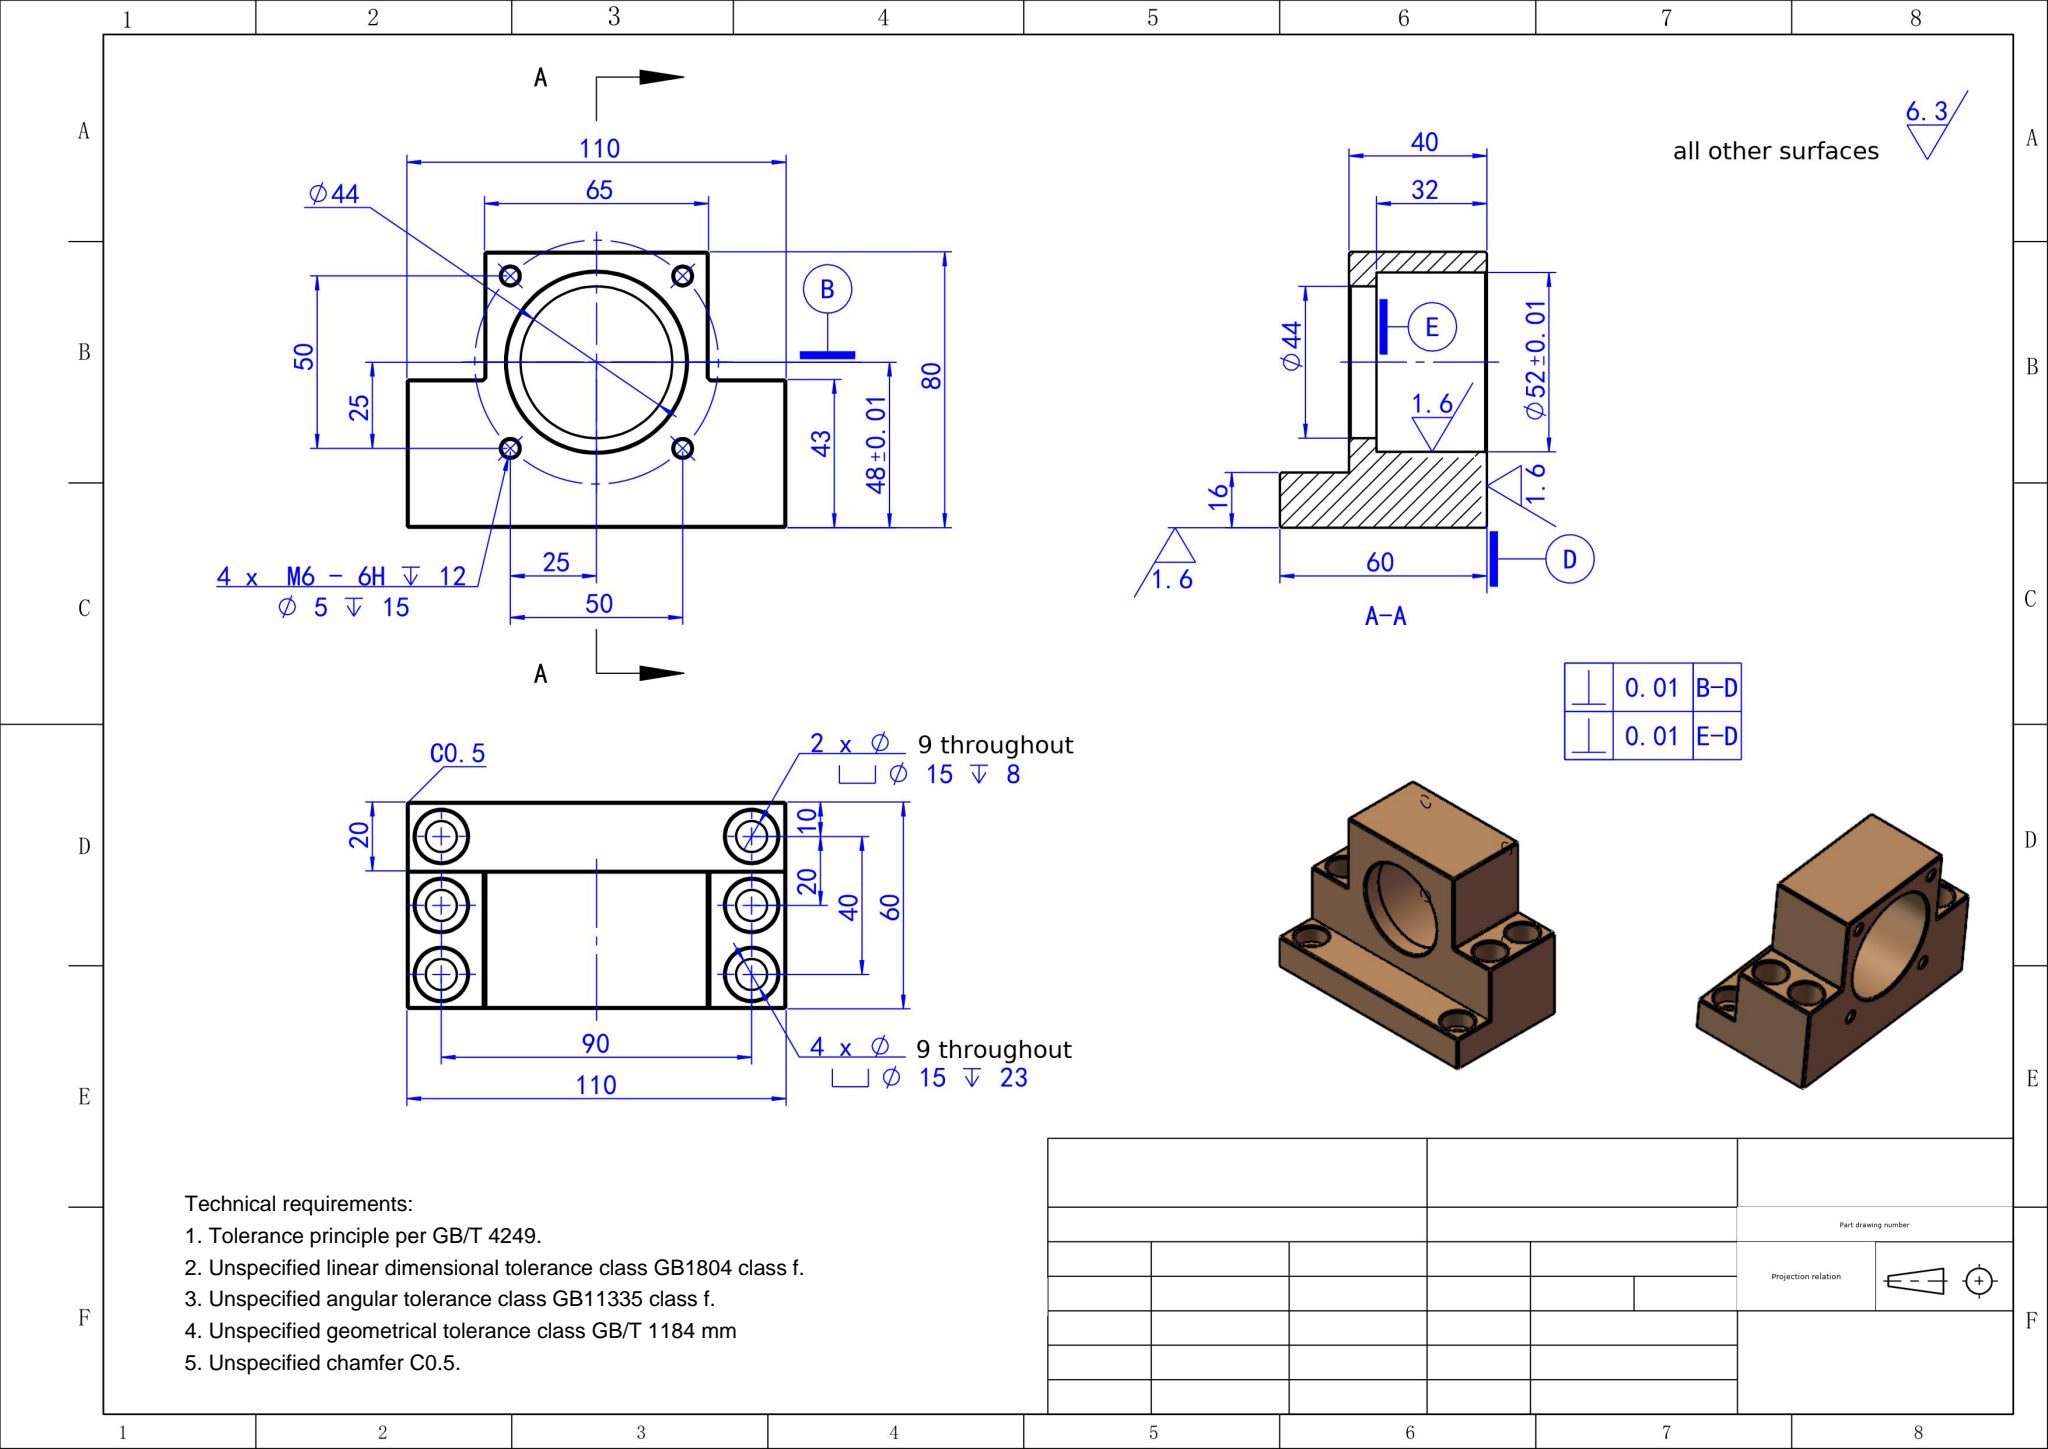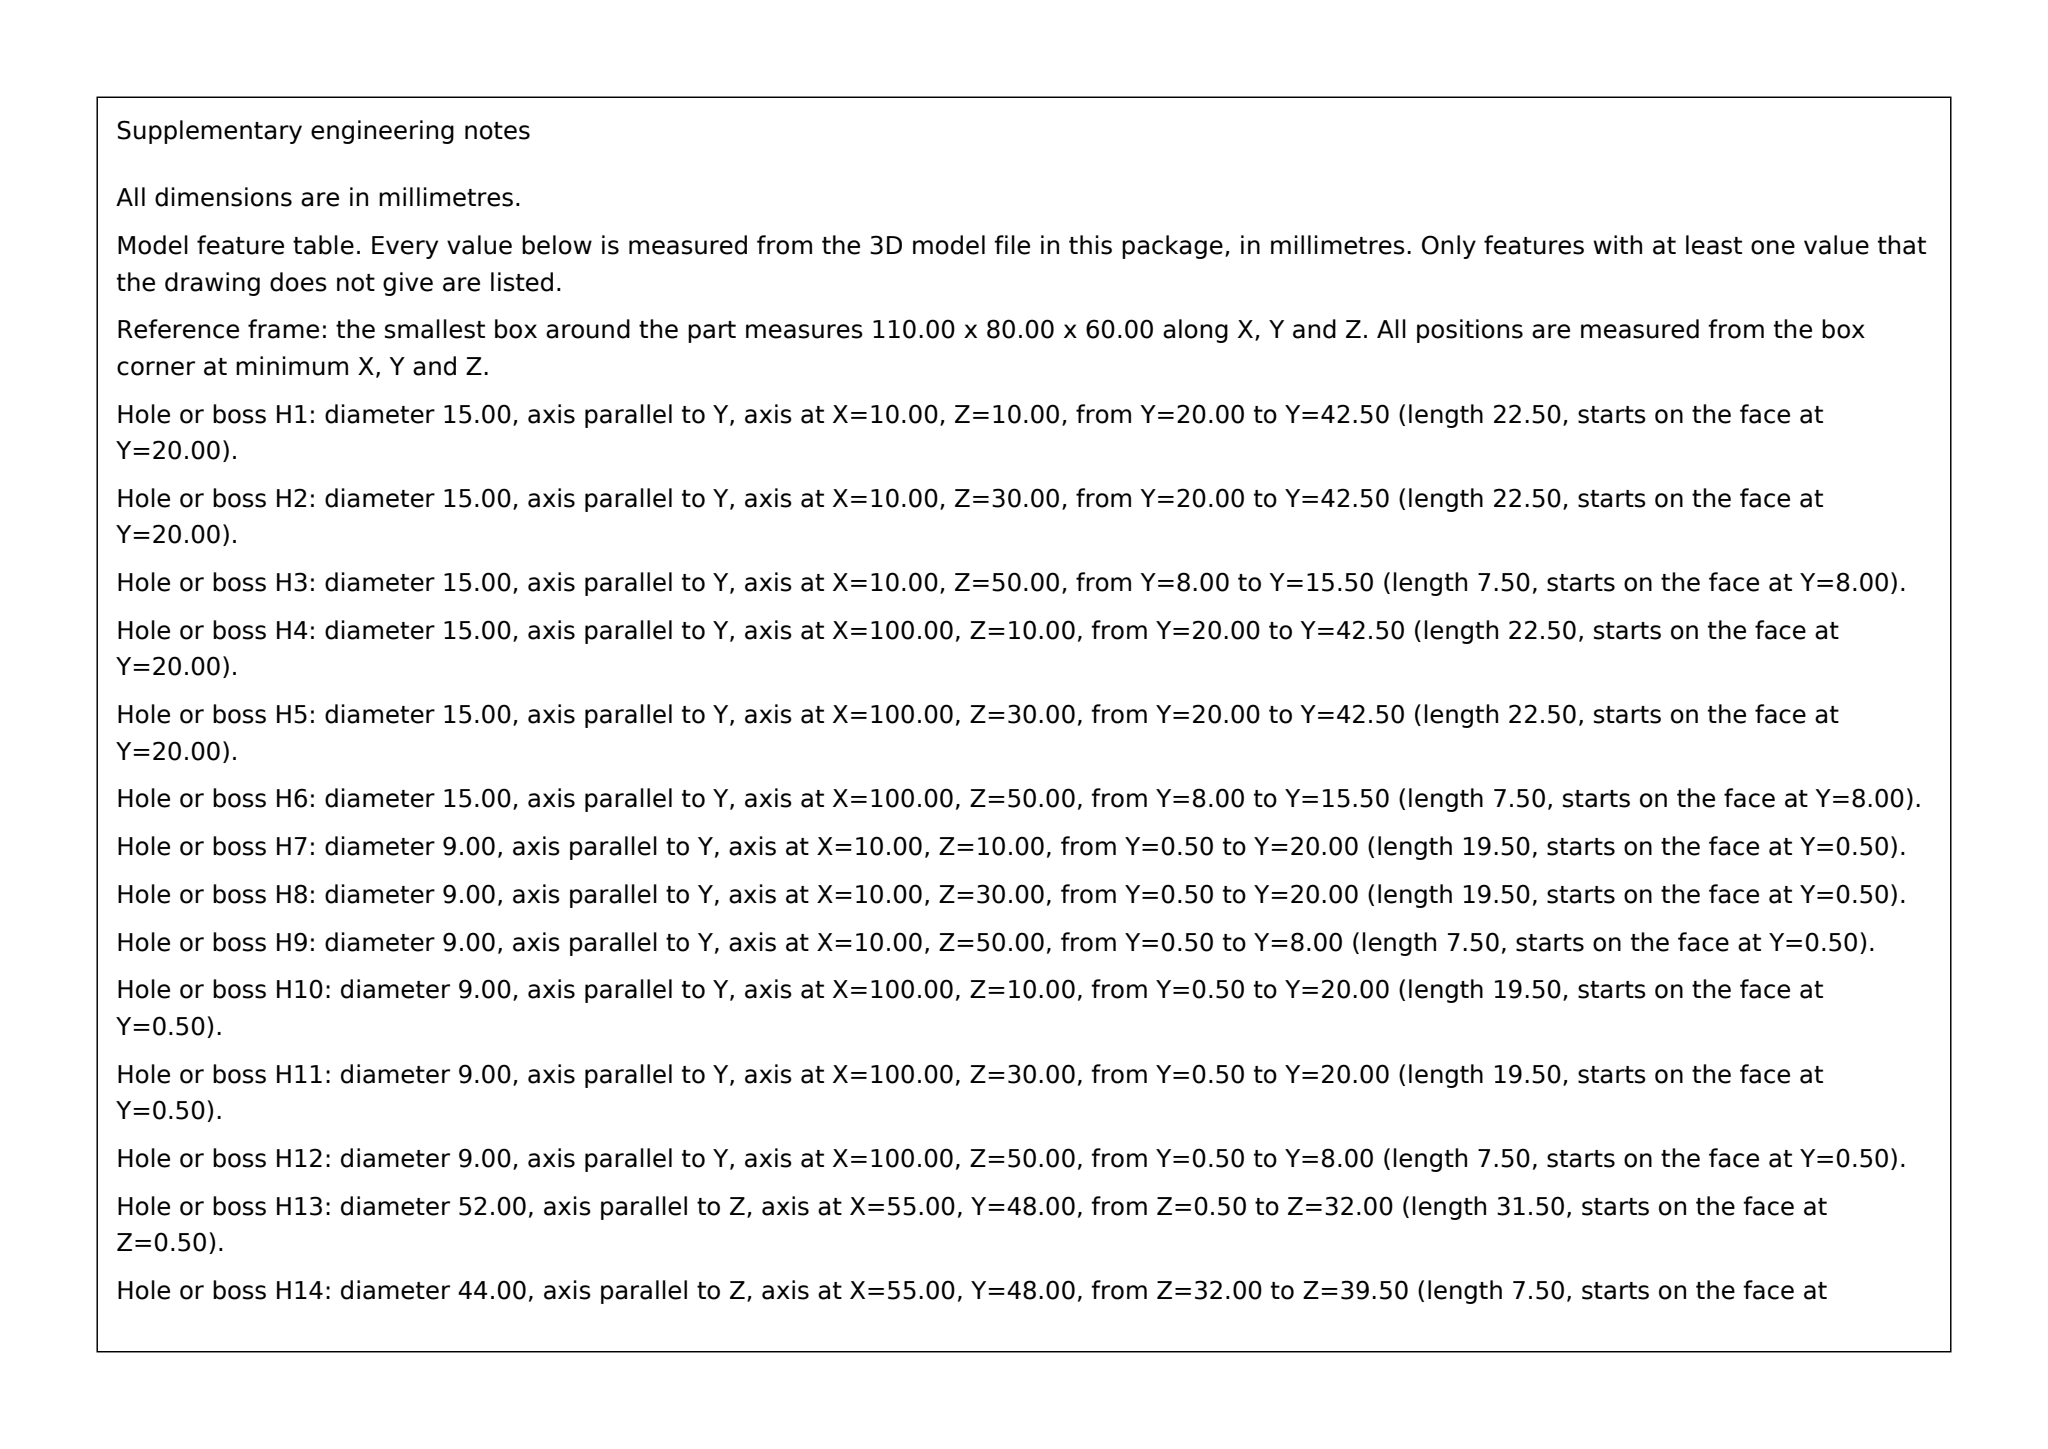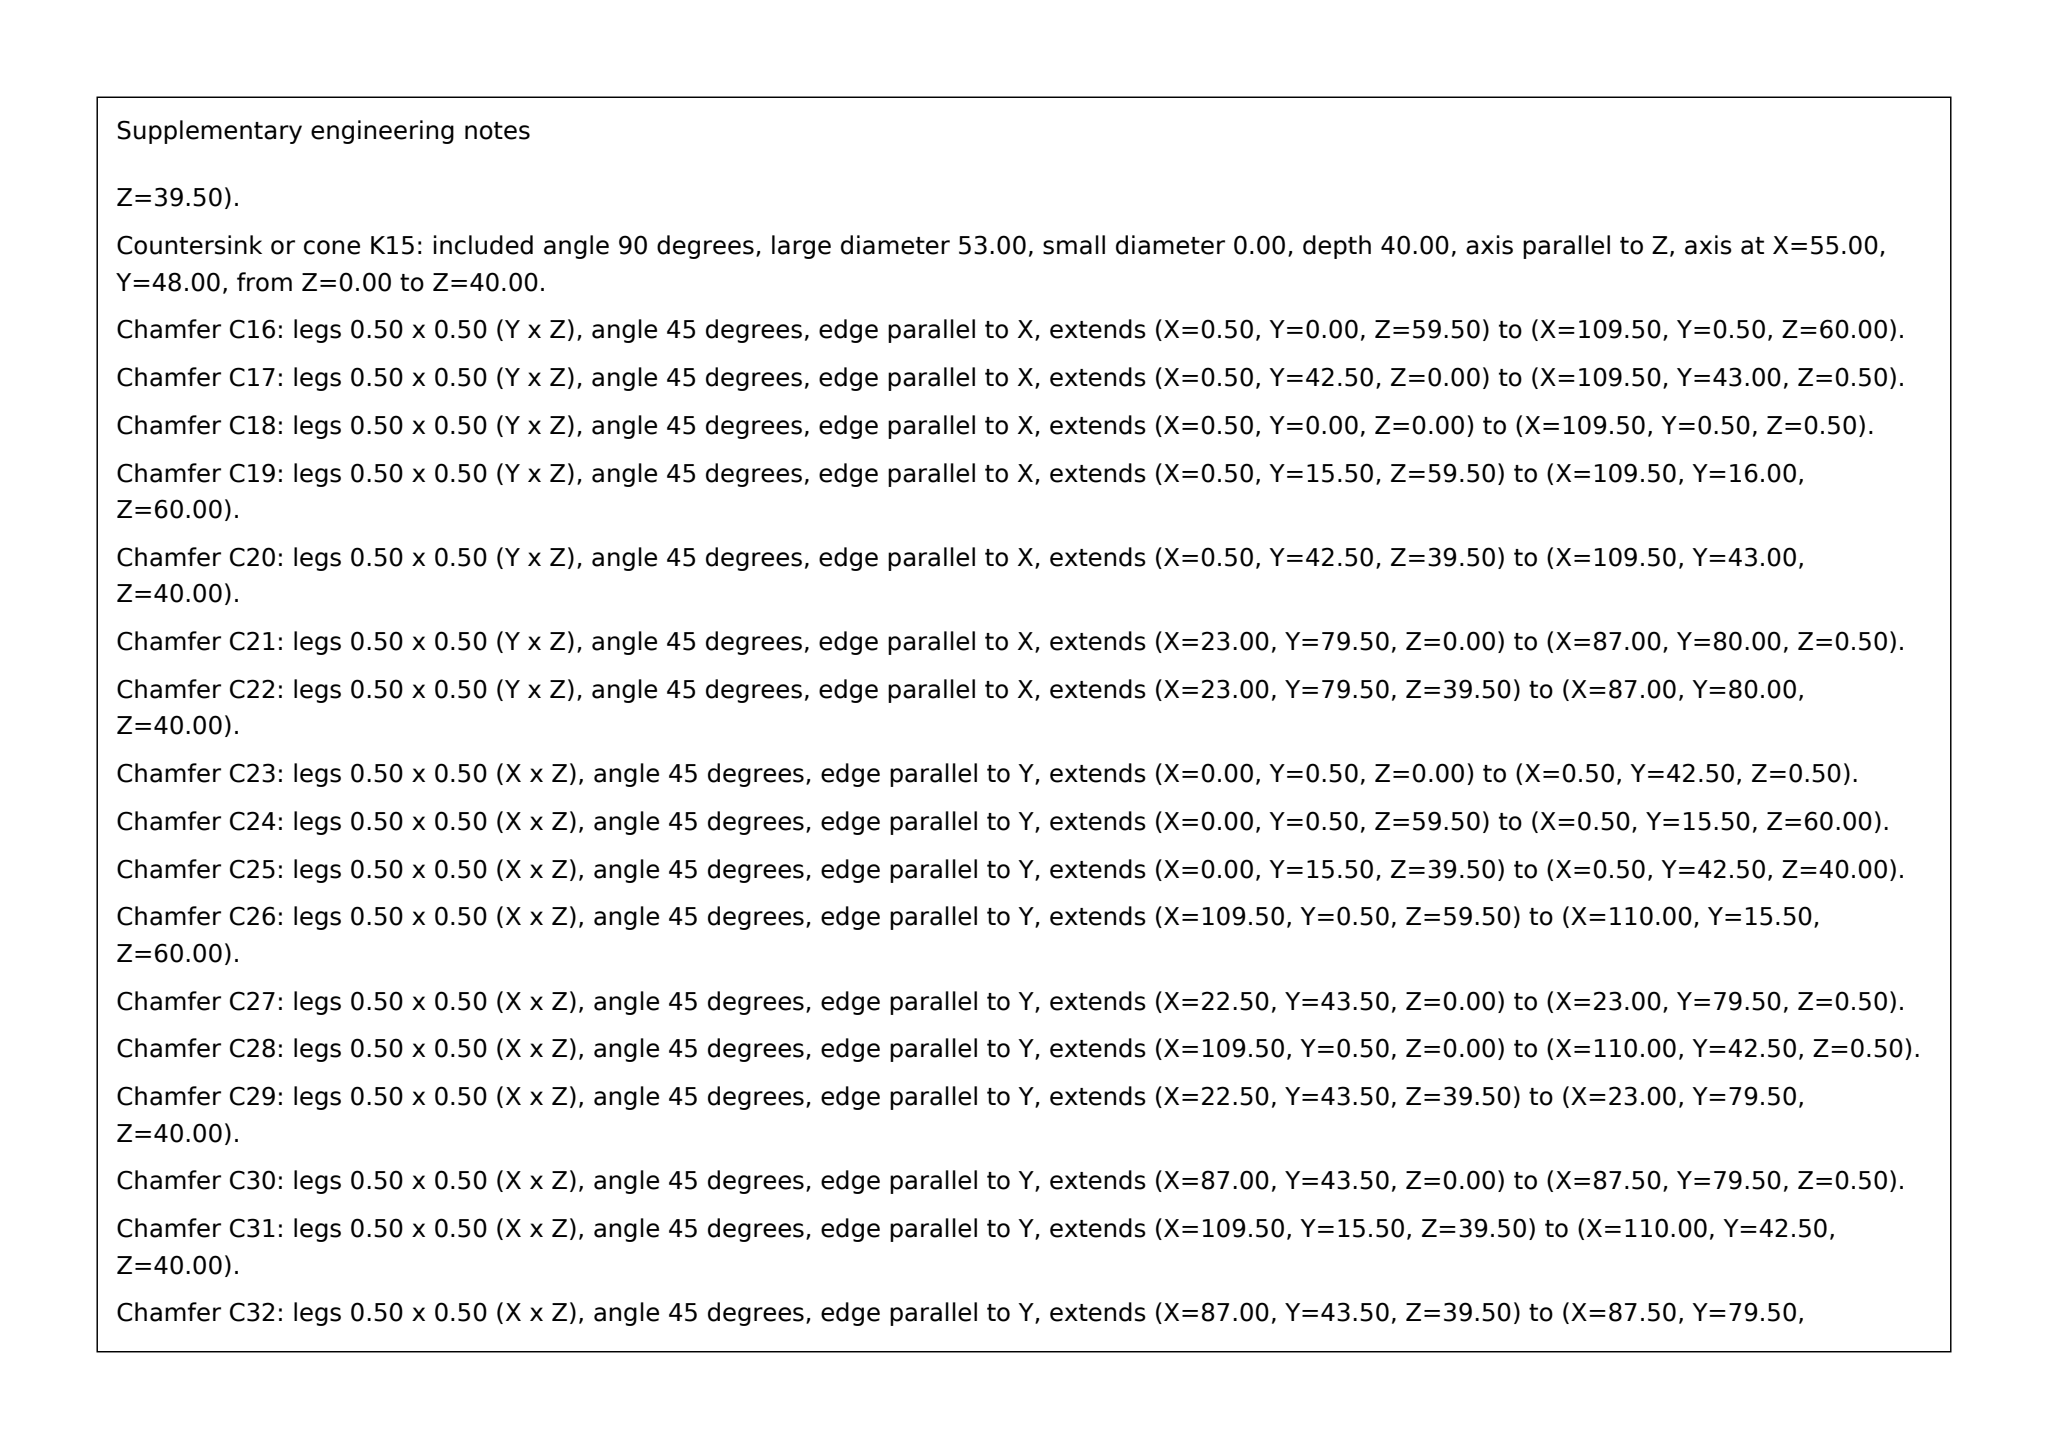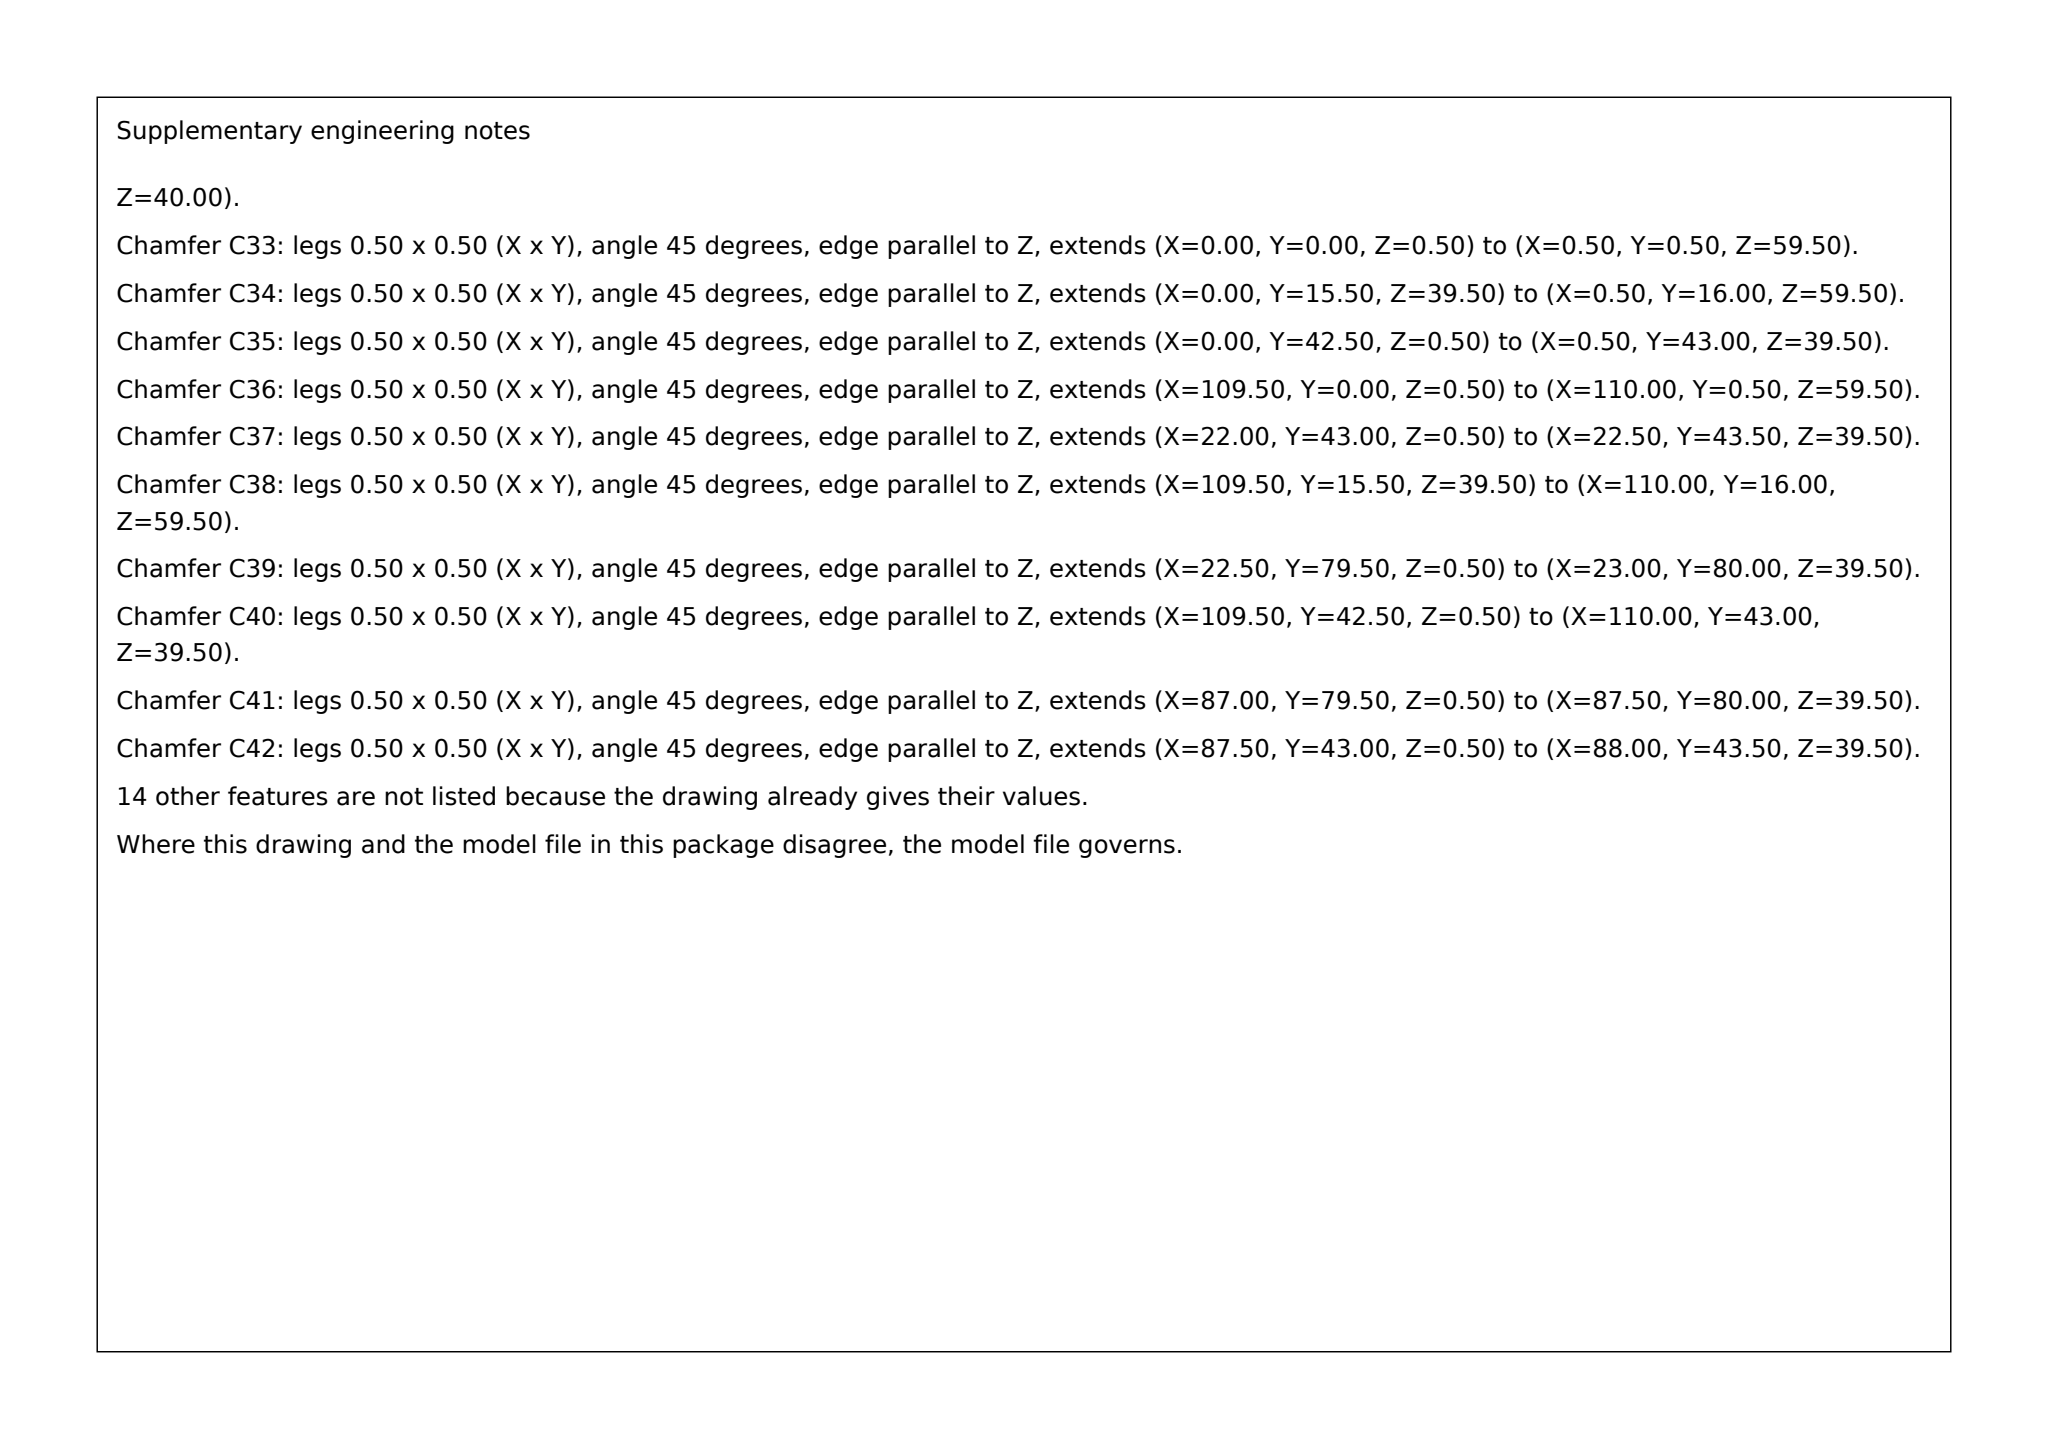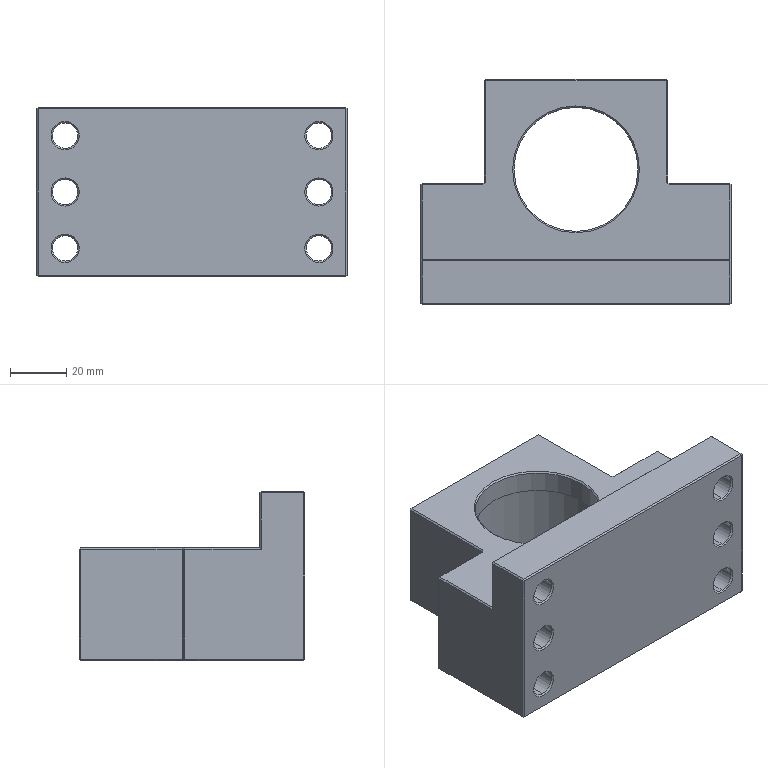Part | SolidWorks | mm | 1 solid | 146 faces | box 110 x 80 x 60 mm | volume 213825 mm3 | plane 66 | cone 44 | cylinder 36 | commonest cylinder face diameters 15 x12 9 x12 5 x8 52 x2 44 x2
build123d program:
from build123d import *

# Parameters (mm, degrees)
SKETCH1_R                                          = 22
BOSS_EXTRUDE1_DEPTH                                = 30
SKETCH2_W                                          = 110
SKETCH2_H                                          = 64
CUT_EXTRUDE1_DEPTH                                 = 20
HOLE_SIZE_ACCORDING_TO_HEXALOBULAR_SOC_D           = 9
HOLE_SIZE_ACCORDING_TO_HEXALOBULAR_SOC_CBORE_D     = 15
HOLE_SIZE_ACCORDING_TO_HEXALOBULAR_SOC_CBORE_DEPTH = 23
HOLE_SIZE_ACCORDING_TO_HEXALOBULAR_2_D             = 9
HOLE_SIZE_ACCORDING_TO_HEXALOBULAR_2_CBORE_D       = 15
HOLE_SIZE_ACCORDING_TO_HEXALOBULAR_2_CBORE_DEPTH   = 8
SKETCH5_R                                          = 26
CUT_EXTRUDE2_DEPTH                                 = 32
CIRPATTERN1_COUNT                                  = 4
CHAMFER1_SIZE                                      = 0.5


with BuildPart() as part:
    # Sketch1 → Boss-Extrude1 (new, symmetric)
    with BuildSketch(Plane.XY):
        Polygon((-55, -5), (-32.5, -5), (-32.5, 32), (32.5, 32), (32.5, -5), (55, -5), (55, -48), (-55, -48), align=None)
        Circle(SKETCH1_R, mode=Mode.SUBTRACT)
    extrude(amount=BOSS_EXTRUDE1_DEPTH, both=True)

    # Sketch2 → Cut-Extrude1 (cut)
    with BuildSketch(Plane.XY.offset(30)):
        Rectangle(SKETCH2_W, SKETCH2_H)
    extrude(amount=-CUT_EXTRUDE1_DEPTH, mode=Mode.SUBTRACT)

    # Hole Size _According to_ Hexalobular Soc (through all)
    with Locations(Plane(origin=(0, -5, 0), x_dir=(1, 0, 0), z_dir=(0, 1, 0))):
        with Locations((-45, 0), (-45, 20), (45, 0), (45, 20)):
            CounterBoreHole(HOLE_SIZE_ACCORDING_TO_HEXALOBULAR_SOC_D / 2, HOLE_SIZE_ACCORDING_TO_HEXALOBULAR_SOC_CBORE_D / 2, HOLE_SIZE_ACCORDING_TO_HEXALOBULAR_SOC_CBORE_DEPTH)

    # Hole Size _According to_ Hexalobular 2 (through all)
    with Locations(Plane(origin=(0, -32, 0), x_dir=(1, 0, 0), z_dir=(0, 1, 0))):
        with Locations((-45, -20), (45, -20)):
            CounterBoreHole(HOLE_SIZE_ACCORDING_TO_HEXALOBULAR_2_D / 2, HOLE_SIZE_ACCORDING_TO_HEXALOBULAR_2_CBORE_D / 2, HOLE_SIZE_ACCORDING_TO_HEXALOBULAR_2_CBORE_DEPTH)

    # Sketch5 → Cut-Extrude2 (cut)
    with BuildSketch(Plane(origin=(0, 0, -30), x_dir=(-1, 0, 0), z_dir=(0, 0, -1))):
        Circle(SKETCH5_R)
    extrude(amount=-CUT_EXTRUDE2_DEPTH, mode=Mode.SUBTRACT)

    # Sketch6 → M6 Tapped Hole1 (revolve, cut)
    with BuildSketch(Plane(origin=(25, -25, -30), x_dir=(0, 1, 0), z_dir=(1, 0, 0))):
        Polygon((0, 0), (0, 16.502), (2.5, 15), (2.5, 0), align=None)
    m6_tapped_hole1 = revolve(axis=Axis((25, -25, -36.35), (0, 0, 1)), mode=Mode.SUBTRACT)

    # CirPattern1: M6 Tapped Hole1 ×4 about axis
    cirpattern1_axis = Axis((0, 0, 0), (0, 0, 1))
    for i in range(1, CIRPATTERN1_COUNT):
        add(m6_tapped_hole1.rotate(cirpattern1_axis, i * 360 / CIRPATTERN1_COUNT), mode=Mode.SUBTRACT)

    # Chamfer1
    chamfer1_edges = [part.edges().sort_by_distance(p)[0] for p in [
        (55, -40, 30),
        (0, -48, -30),
        (26, 0, -30),
        (-55, -26.5, -30),
        (25, -27.5, -30),
        (-27.5, -25, -30),
        (-25, 27.5, -30),
        (27.5, 25, -30),
        (55, -48, 0),
        (-55, -48, 0),
        (-55, -5, -10),
        (-32.5, -5, -10),
        (-32.5, 32, -10),
        (32.5, 32, -10),
        (32.5, -5, -10),
        (55, -5, -10),
        (-55, -40, 30),
        (55, -18.5, 10),
        (0, 32, 10),
        (-55, -18.5, 10),
        (-55, -32, 20),
        (32.5, 13.5, 10),
        (43.75, -5, 10),
        (-43.75, -5, 10),
        (-32.5, 13.5, 10),
        (-22, 0, 10),
        (0, -32, 30),
        (55, -32, 20),
        (37.5, -5, -20),
        (49.5, -48, -20),
        (37.5, -5, 0),
        (49.5, -48, 0),
        (0, -48, 30),
        (-52.5, -5, -20),
        (-40.5, -48, -20),
        (-43.75, -5, -30),
        (-52.5, -5, 0),
        (-40.5, -48, 0),
        (-32.5, 13.5, -30),
        (0, 32, -30),
        (37.5, -32, 20),
        (49.5, -48, 20),
        (32.5, 13.5, -30),
        (43.75, -5, -30),
        (-52.5, -32, 20),
        (-40.5, -48, 20),
        (55, -26.5, -30),
    ]]
    chamfer(chamfer1_edges, length=CHAMFER1_SIZE)


solid = part.part